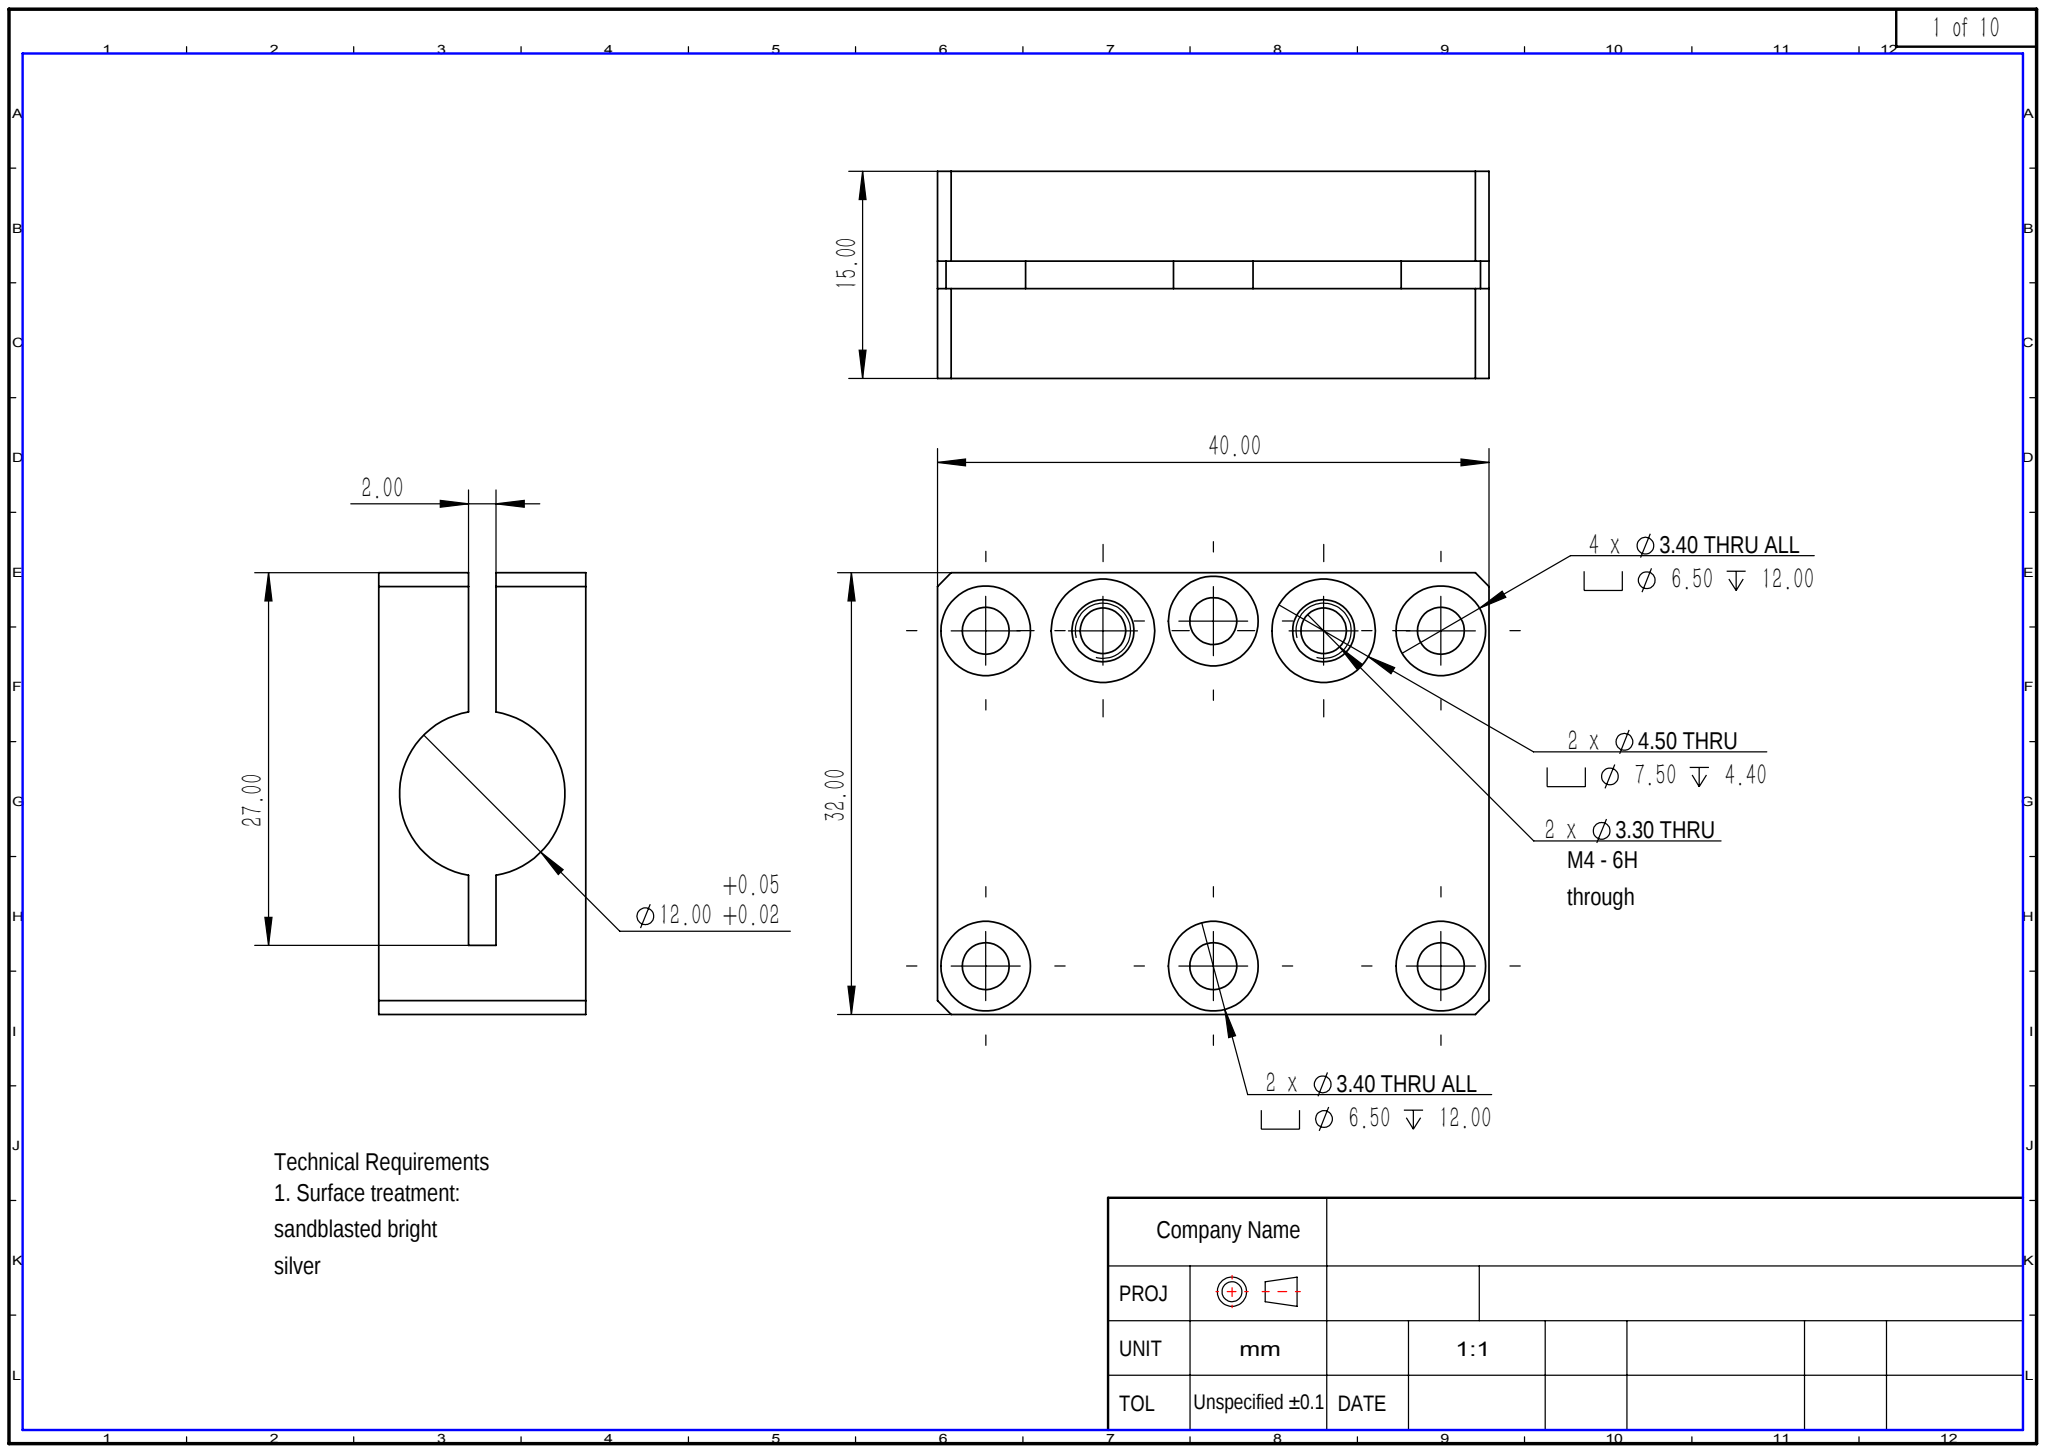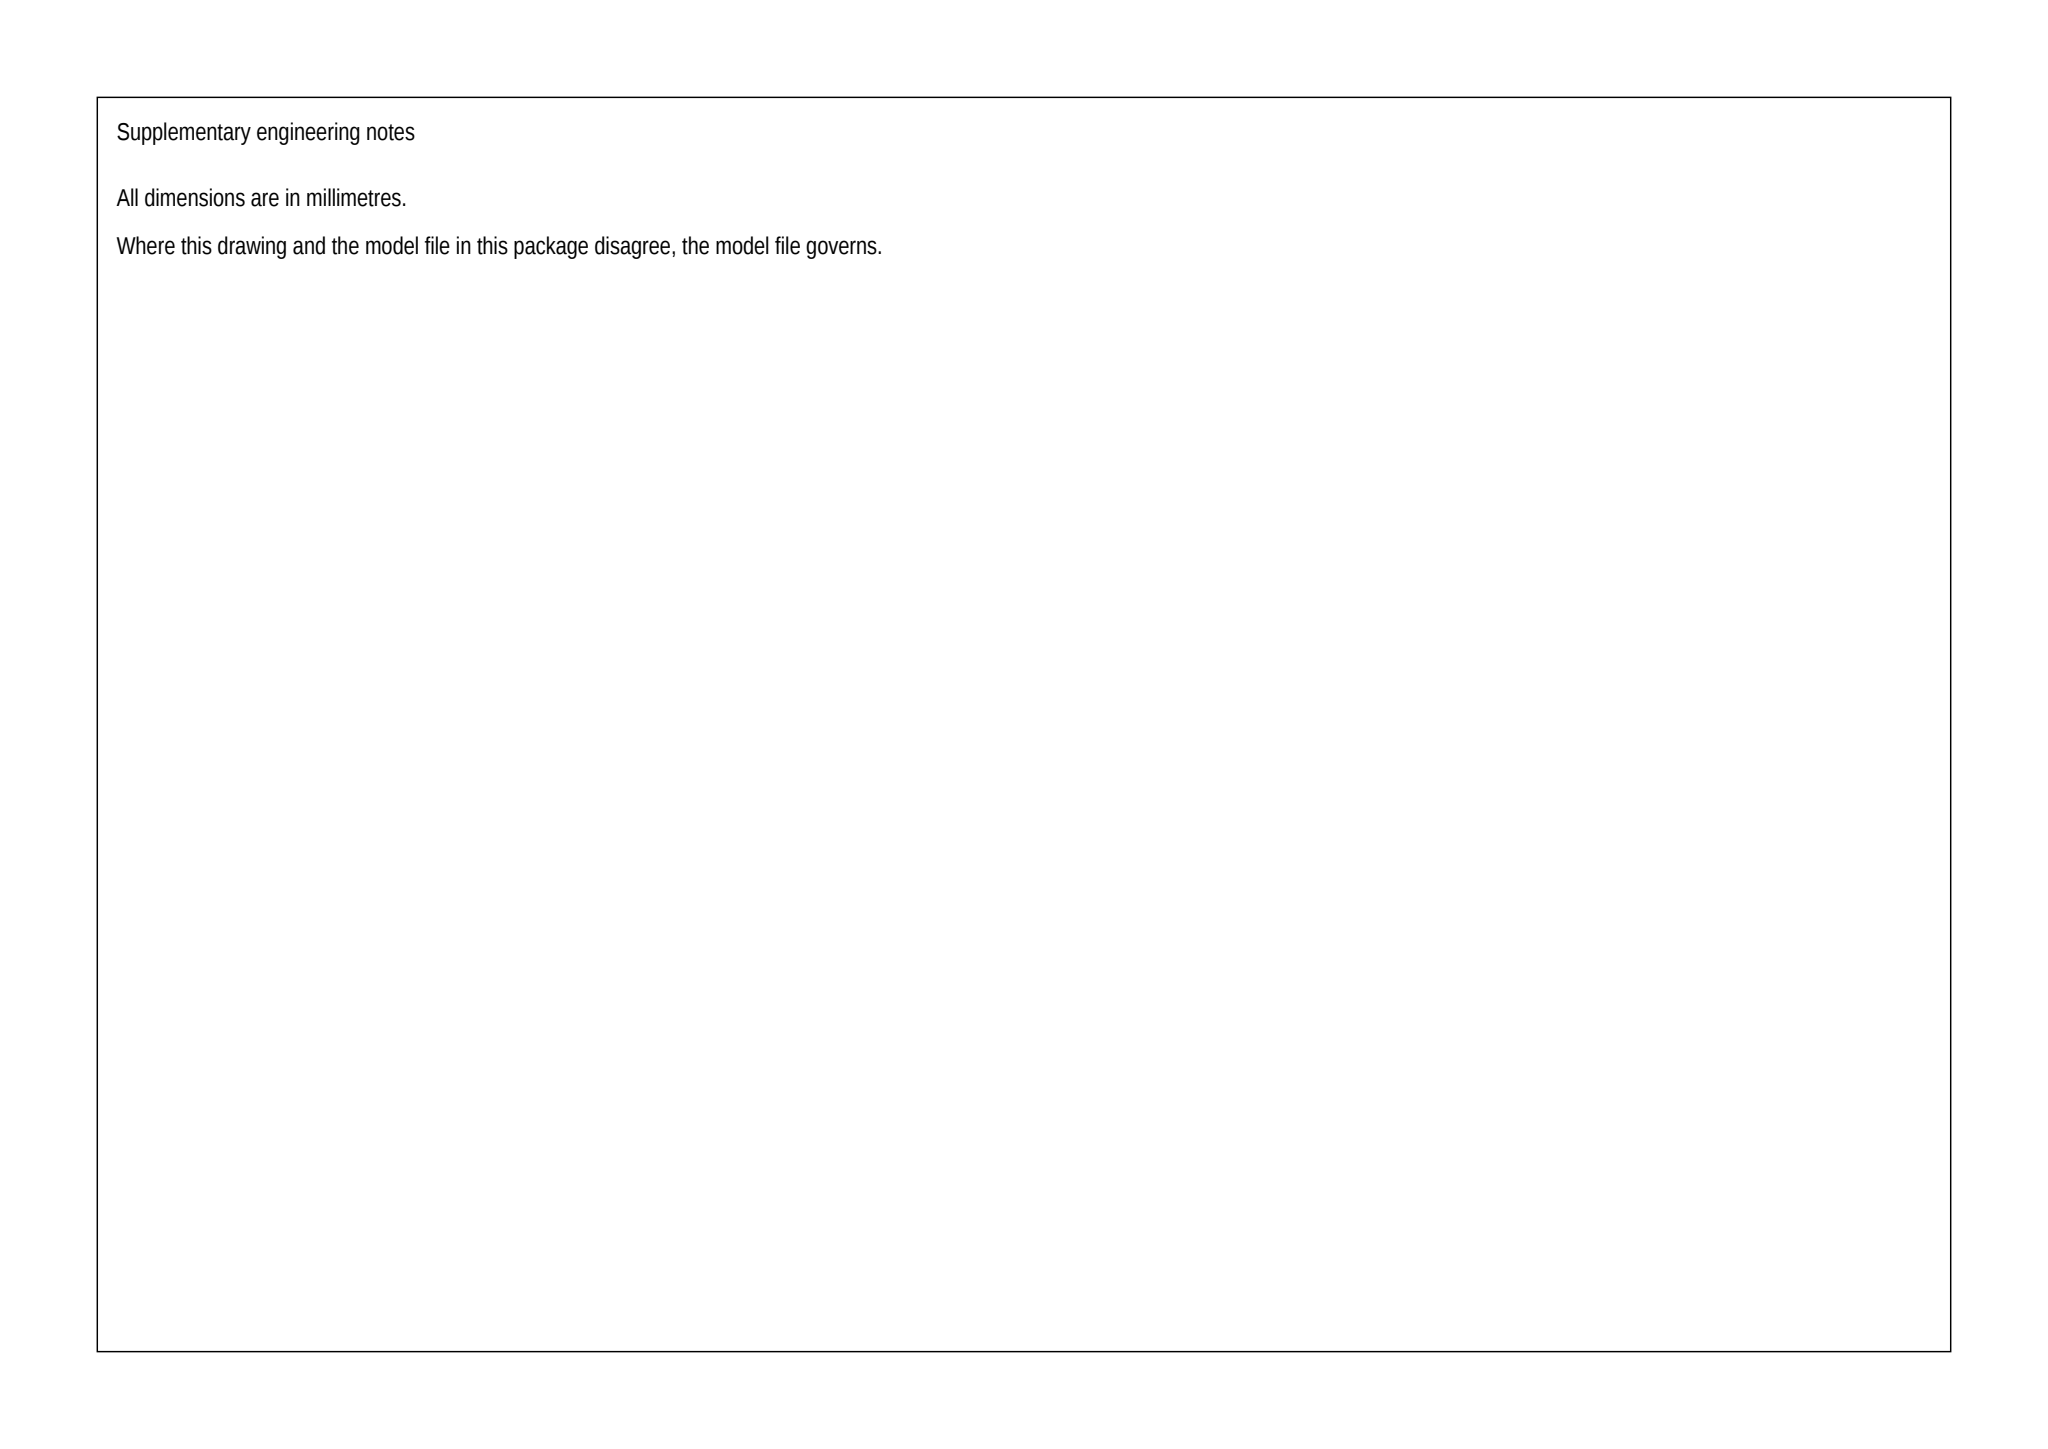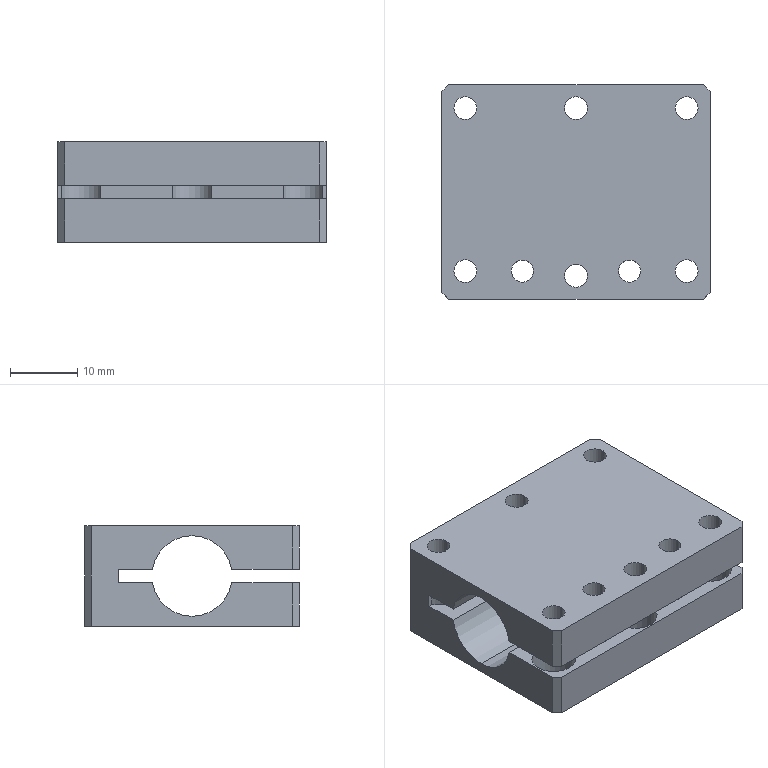Part | SolidWorks | mm | 1 solid | 74 faces | box 40 x 32 x 15 mm | volume 10567 mm3 | cylinder 45 | plane 29 | commonest cylinder face diameters 6.5 x18 3.4 x12 3.3 x4 7.5 x4 4.5 x4 12 x3
Drawing notes:
Ø12 BORE THRU, 40.00 LG; CL 16.00 FROM TOP EDGE, 7.50 FROM EA FACE | from the solid: Ø12 x-axis cyl at y=16.0, z=7.5, length 40.0 = bbox x; bbox 40x32x15
2.00 SLOT CL ON BORE, Z 6.50-8.50, FULL 40.00 LG, 10.00 DP FROM TOP FACE | from the solid: z planes at 6.50 (2) & 8.50 (2) about z=7.5; y=0 face split by slot; bore top y=16-6=10
LOWER RELIEF NOTCH 2.00 W x 5.00 DP, Z 6.50-8.50, FULL 40.00 LG | from the solid: notch from bore (y=22) to y planes at 27.0 (4); z 6.5-8.5; spans 40.0
4X Ø3.40 CBORE: X 3.50 & 36.50, Y 4.20 & 28.50 FROM TOP LH CORNER | from the solid: Ø3.4 z-holes at (3.5,4.2),(36.5,4.2),(3.5,28.5),(36.5,28.5); bbox 40x32
2X Ø3.40 CBORE: X 20.00 CL, Y 3.50 & 28.50 FROM TOP LH CORNER | from the solid: Ø3.4 z-holes at (20.0,3.5) and (20.0,28.5); X CL = 40/2; 32-28.5=3.5
2X Ø4.50 W/ Ø7.50 CBORE: X 12.00 & 28.00, Y 4.20 FROM TOP LH CORNER | from the solid: Ø4.5 & Ø7.5 z-cyls at (12.0,4.2) and (28.0,4.2)
2X Ø3.30 M4-6H COAX W/ Ø4.50: X 12.00 & 28.00, Y 4.20 FROM TOP LH CORNER | from the solid: Ø3.3 z-cyls at (12.0,4.2) and (28.0,4.2), same axes as Ø4.5/Ø7.5
ALL PERIMETER EDGES SHARP AS MODELED: NO CHAMFERS OR FILLETS ARE DEFINED ON THE 40.00 x 32.00 x 15.00 BLOCK; BREAK EDGES ONLY AS REQUIRED TO REMOVE BURRS. | from the solid: cones[included_angle,ref_dia] is empty and fillet_radii is empty; bbox_xyz [40.0, 32.0, 15.0] with only planar faces at x=0/40, y=0/27/32, z=0/4.4/6.5/8.5/12/15
CBORE ENTRY FACE: ALL 6X Ø6.50 CBORES ARE MACHINED FROM THE Z=0.00 FACE (FACE OPPOSITE THE 15.00 TOP FACE), 12.00 DEEP TO A FLAT BOTTOM AT Z=12.00; Ø3.40 CONTINUES THE REMAINING 3.00 THRU TO THE TOP FACE. LOCATIONS X 3.50/20.00/36.50, Y 3.50 & 28.50 (Y 4.20 AT X 3.50, 36.50) FROM MIN CORNER. | from the solid: cylinders[6.5,z,(3.5/20.0/36.5, 4.2/3.5/28.5),12.0] and split 6.5+3.5 segments, bottoms at axis_plane z=12.0 (count 6); cylinders[3.4,z,same XY,3.0] spanning z=12.0 to 15.0
2X Ø7.50 CBORE 4.40 DEEP (CLAMP SCREW) ALSO ENTERED FROM THE SAME Z=0.00 FACE AT X 12.00 & 28.00, Y 4.20 FROM MIN CORNER; Ø4.50 CONTINUES FROM Z=4.40 TO Z=6.50, AND THE M4-6H (Ø3.30) TAPPED PORTION RUNS Z=8.50 TO 15.00 COAXIAL, INTERRUPTED BY THE 2.00 WIDE RELIEF AT Z 6.50-8.50. | from the solid: cylinders[7.5,z,(12.0/28.0,4.2),4.4] with axis_plane z=4.4 (count 2); cylinders[4.5,z,same,2.1] (z4.4-6.5); cylinders[3.3,z,same,6.5] (z8.5-15.0); axis_planes z=6.5 and z=8.5
build123d program:
from build123d import *

# Parameters (mm, degrees)
SKETCH1_W                                       = 40
SKETCH1_H                                       = 32
BOSS_EXTRUDE1_DEPTH                             = 7.5
SKETCH2_R                                       = 6
CUT_EXTRUDE1_DEPTH                              = 44.729
SKETCH3_W                                       = 2
SKETCH3_H                                       = 27
CUT_EXTRUDE2_DEPTH                              = 44.729
M3_HEX_SOCKET_HEAD_CAP_SCREW_CBORE1_D           = 3.4
M3_HEX_SOCKET_HEAD_CAP_SCREW_CBORE1_CBORE_D     = 6.5
M3_HEX_SOCKET_HEAD_CAP_SCREW_CBORE1_CBORE_DEPTH = 12
M3_HEX_SOCKET_HEAD_CAP_SCREW_CBORE2_D           = 3.4
M3_HEX_SOCKET_HEAD_CAP_SCREW_CBORE2_CBORE_D     = 6.5
M3_HEX_SOCKET_HEAD_CAP_SCREW_CBORE2_CBORE_DEPTH = 12
M4_HEX_SOCKET_HEAD_CAP_SCREW_CBORE1_D           = 4.5
M4_HEX_SOCKET_HEAD_CAP_SCREW_CBORE1_DEPTH       = 6.5
M4_HEX_SOCKET_HEAD_CAP_SCREW_CBORE1_CBORE_D     = 7.5
M4_HEX_SOCKET_HEAD_CAP_SCREW_CBORE1_CBORE_DEPTH = 4.4
M4_TAPPED_HOLE1_D                               = 3.3
CHAMFER1_SIZE                                   = 1


with BuildPart() as part:
    # Sketch1 → Boss-Extrude1 (new, symmetric)
    with BuildSketch(Plane.XY):
        Rectangle(SKETCH1_W, SKETCH1_H)
    extrude(amount=BOSS_EXTRUDE1_DEPTH, both=True)

    # Sketch2 → Cut-Extrude1 (cut, through all)
    with BuildSketch(Plane(origin=(20, 0, 0), x_dir=(0, 0, -1), z_dir=(1, 0, 0))):
        Circle(SKETCH2_R)
    extrude(amount=-CUT_EXTRUDE1_DEPTH, mode=Mode.SUBTRACT)

    # Sketch3 → Cut-Extrude2 (cut, through all)
    with BuildSketch(Plane(origin=(20, 0, 0), x_dir=(0, 0, -1), z_dir=(1, 0, 0))):
        with Locations((0, -2.5)):
            Rectangle(SKETCH3_W, SKETCH3_H)
    extrude(amount=-CUT_EXTRUDE2_DEPTH, mode=Mode.SUBTRACT)

    # M3 Hex Socket Head Cap Screw CBORE1 (through all)
    with Locations(Plane(origin=(0, 0, -7.5), x_dir=(-1, 0, 0), z_dir=(0, 0, -1))):
        with Locations((16.5, 12.5), (-16.5, -11.8)):
            m3_hex_socket_head_cap_screw_cbore1 = CounterBoreHole(M3_HEX_SOCKET_HEAD_CAP_SCREW_CBORE1_D / 2, M3_HEX_SOCKET_HEAD_CAP_SCREW_CBORE1_CBORE_D / 2, M3_HEX_SOCKET_HEAD_CAP_SCREW_CBORE1_CBORE_DEPTH)

    # Mirror1: M3 Hex Socket Head Cap Screw CBORE1 across plane
    add(m3_hex_socket_head_cap_screw_cbore1.mirror(Plane(origin=(0, 0, 0), x_dir=(0, 0, 1), z_dir=(1, 0, 0))), mode=Mode.SUBTRACT)

    # M3 Hex Socket Head Cap Screw CBORE2 (through all)
    with Locations(Plane(origin=(0, 0, -7.5), x_dir=(-1, 0, 0), z_dir=(0, 0, -1))):
        with Locations((0, 12.5), (0, -12.5)):
            CounterBoreHole(M3_HEX_SOCKET_HEAD_CAP_SCREW_CBORE2_D / 2, M3_HEX_SOCKET_HEAD_CAP_SCREW_CBORE2_CBORE_D / 2, M3_HEX_SOCKET_HEAD_CAP_SCREW_CBORE2_CBORE_DEPTH)

    # M4 Hex Socket Head Cap Screw CBORE1
    with Locations(Plane(origin=(0, 0, -7.5), x_dir=(-1, 0, 0), z_dir=(0, 0, -1))):
        with Locations((-8, -11.8), (8, -11.8)):
            CounterBoreHole(M4_HEX_SOCKET_HEAD_CAP_SCREW_CBORE1_D / 2, M4_HEX_SOCKET_HEAD_CAP_SCREW_CBORE1_CBORE_D / 2, M4_HEX_SOCKET_HEAD_CAP_SCREW_CBORE1_CBORE_DEPTH, depth=M4_HEX_SOCKET_HEAD_CAP_SCREW_CBORE1_DEPTH)

    # M4 Tapped Hole1 (through all)
    with Locations(Plane(origin=(0, 0, 1), x_dir=(-1, 0, 0), z_dir=(0, 0, -1))):
        with Locations((-8, -11.8), (8, -11.8)):
            Hole(M4_TAPPED_HOLE1_D / 2)

    # Chamfer1
    chamfer1_edges = [part.edges().sort_by_distance(p)[0] for p in [
        (20, -16, -4.25),
        (-20, -16, -4.25),
        (20, -16, 4.25),
        (-20, -16, 4.25),
        (-20, 16, 0),
        (20, 16, 0),
    ]]
    chamfer(chamfer1_edges, length=CHAMFER1_SIZE)


solid = part.part